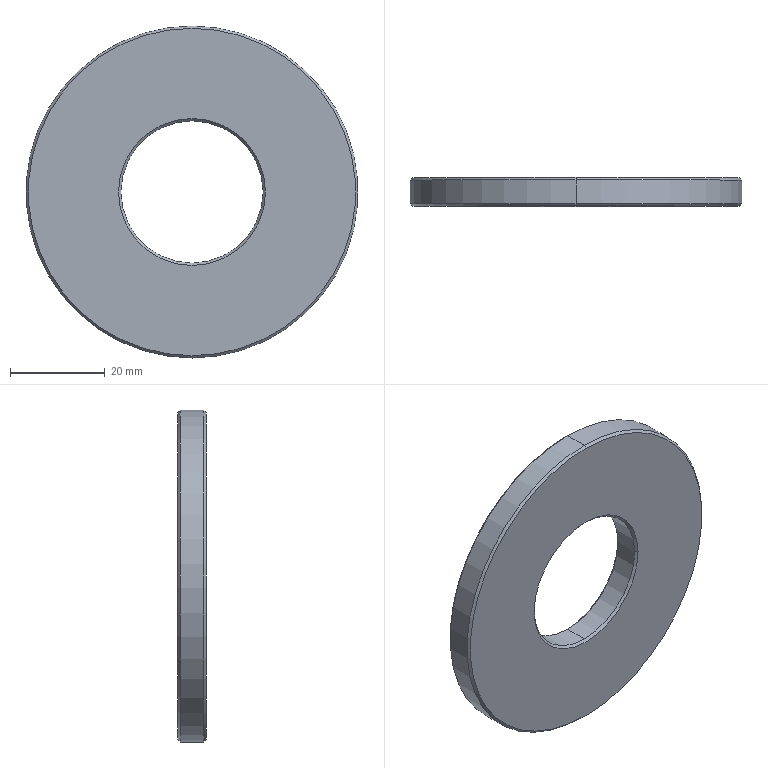Component | SolidWorks | YC1-250-04BalancerAssembly#16673-1_YC1-250-04-08Washer-1 | 1 solid | 14 faces | box 70 x 6 x 70 mm | volume 18771 mm3 | cone 8 | cylinder 4 | plane 2 | commonest cylinder face diameters 30 x2 70 x2 | material Plain Carbon Steel
STEP:
#1=COLOUR_RGB('',0.7922,0.8196,0.9333);
#2=FILL_AREA_STYLE_COLOUR('',#1);
#3=FILL_AREA_STYLE('',(#2));
#4=SURFACE_STYLE_FILL_AREA(#3);
#5=SURFACE_SIDE_STYLE('',(#4));
#6=SURFACE_STYLE_USAGE(.BOTH.,#5);
#7=PRESENTATION_STYLE_ASSIGNMENT((#6));
#8=CARTESIAN_POINT('',(-18.11,165.573,-0.5906));
#9=VERTEX_POINT('',#8);
#10=CARTESIAN_POINT('',(-18.11,165.573,0.5906));
#11=VERTEX_POINT('',#10);
#12=CARTESIAN_POINT('',(-18.11,165.573,-0.));
#13=DIRECTION('',(0.,1.,0.));
#14=DIRECTION('',(0.,0.,1.));
#15=AXIS2_PLACEMENT_3D('',#12,#13,#14);
#16=CIRCLE('',#15,0.5906);
#17=EDGE_CURVE('',#9,#11,#16,.T.);
#18=ORIENTED_EDGE('',*,*,#17,.F.);
#19=CARTESIAN_POINT('',(-18.11,165.592,-0.6102));
#20=VERTEX_POINT('',#19);
#21=CARTESIAN_POINT('',(-18.11,165.592,-0.6102));
#22=DIRECTION('',(0.,0.7071,-0.7071));
#23=VECTOR('',#22,39.37);
#24=LINE('',#21,#23);
#25=EDGE_CURVE('',#9,#20,#24,.T.);
#26=ORIENTED_EDGE('',*,*,#25,.T.);
#27=CARTESIAN_POINT('',(-18.11,165.592,0.6102));
#28=VERTEX_POINT('',#27);
#29=CARTESIAN_POINT('',(-18.11,165.592,-0.));
#30=DIRECTION('',(0.,-1.,0.));
#31=DIRECTION('',(0.,0.,1.));
#32=AXIS2_PLACEMENT_3D('',#29,#30,#31);
#33=CIRCLE('',#32,0.6102);
#34=EDGE_CURVE('',#28,#20,#33,.T.);
#35=ORIENTED_EDGE('',*,*,#34,.F.);
#36=CARTESIAN_POINT('',(-18.11,165.592,0.6102));
#37=DIRECTION('',(0.,0.7071,0.7071));
#38=VECTOR('',#37,39.37);
#39=LINE('',#36,#38);
#40=EDGE_CURVE('',#11,#28,#39,.T.);
#41=ORIENTED_EDGE('',*,*,#40,.F.);
#42=EDGE_LOOP('',(#18,#26,#35,#41));
#43=FACE_OUTER_BOUND('',#42,.T.);
#44=CARTESIAN_POINT('',(-18.11,165.592,-0.));
#45=DIRECTION('',(0.,1.,0.));
#46=DIRECTION('',(0.,0.,1.));
#47=AXIS2_PLACEMENT_3D('',#44,#45,#46);
#48=CONICAL_SURFACE('',#47,0.6102,0.7854);
#49=ADVANCED_FACE('',(#43),#48,.F.);
#50=CARTESIAN_POINT('',(-18.11,165.592,1.358));
#51=VERTEX_POINT('',#50);
#52=CARTESIAN_POINT('',(-18.11,165.592,-1.358));
#53=VERTEX_POINT('',#52);
#54=CARTESIAN_POINT('',(-18.11,165.592,-0.));
#55=DIRECTION('',(0.,1.,0.));
#56=DIRECTION('',(0.,0.,-1.));
#57=AXIS2_PLACEMENT_3D('',#54,#55,#56);
#58=CIRCLE('',#57,1.358);
#59=EDGE_CURVE('',#51,#53,#58,.T.);
#60=ORIENTED_EDGE('',*,*,#59,.F.);
#61=CARTESIAN_POINT('',(-18.11,165.573,1.378));
#62=VERTEX_POINT('',#61);
#63=CARTESIAN_POINT('',(-18.11,165.573,1.378));
#64=DIRECTION('',(0.,-0.7071,0.7071));
#65=VECTOR('',#64,39.37);
#66=LINE('',#63,#65);
#67=EDGE_CURVE('',#51,#62,#66,.T.);
#68=ORIENTED_EDGE('',*,*,#67,.T.);
#69=CARTESIAN_POINT('',(-18.11,165.573,-1.378));
#70=VERTEX_POINT('',#69);
#71=CARTESIAN_POINT('',(-18.11,165.573,-0.));
#72=DIRECTION('',(0.,1.,0.));
#73=DIRECTION('',(0.,0.,-1.));
#74=AXIS2_PLACEMENT_3D('',#71,#72,#73);
#75=CIRCLE('',#74,1.378);
#76=EDGE_CURVE('',#62,#70,#75,.T.);
#77=ORIENTED_EDGE('',*,*,#76,.T.);
#78=CARTESIAN_POINT('',(-18.11,165.573,-1.378));
#79=DIRECTION('',(0.,-0.7071,-0.7071));
#80=VECTOR('',#79,39.37);
#81=LINE('',#78,#80);
#82=EDGE_CURVE('',#53,#70,#81,.T.);
#83=ORIENTED_EDGE('',*,*,#82,.F.);
#84=EDGE_LOOP('',(#60,#68,#77,#83));
#85=FACE_OUTER_BOUND('',#84,.T.);
#86=CARTESIAN_POINT('',(-18.11,165.573,-0.));
#87=DIRECTION('',(0.,-1.,0.));
#88=DIRECTION('',(0.,0.,-1.));
#89=AXIS2_PLACEMENT_3D('',#86,#87,#88);
#90=CONICAL_SURFACE('',#89,1.378,0.7854);
#91=ADVANCED_FACE('',(#85),#90,.T.);
#92=ORIENTED_EDGE('',*,*,#17,.T.);
#93=CARTESIAN_POINT('',(-18.11,165.376,0.5906));
#94=VERTEX_POINT('',#93);
#95=CARTESIAN_POINT('',(-18.11,165.592,0.5906));
#96=DIRECTION('',(0.,-1.,0.));
#97=VECTOR('',#96,39.37);
#98=LINE('',#95,#97);
#99=EDGE_CURVE('',#11,#94,#98,.T.);
#100=ORIENTED_EDGE('',*,*,#99,.T.);
#101=CARTESIAN_POINT('',(-18.701,165.376,-0.));
#102=VERTEX_POINT('',#101);
#103=CARTESIAN_POINT('',(-18.11,165.376,-0.));
#104=DIRECTION('',(0.,1.,0.));
#105=DIRECTION('',(0.,0.,-1.));
#106=AXIS2_PLACEMENT_3D('',#103,#104,#105);
#107=CIRCLE('',#106,0.5906);
#108=EDGE_CURVE('',#102,#94,#107,.T.);
#109=ORIENTED_EDGE('',*,*,#108,.F.);
#110=CARTESIAN_POINT('',(-18.11,165.376,-0.5906));
#111=VERTEX_POINT('',#110);
#112=CARTESIAN_POINT('',(-18.11,165.376,-0.));
#113=DIRECTION('',(0.,1.,0.));
#114=DIRECTION('',(0.,0.,-1.));
#115=AXIS2_PLACEMENT_3D('',#112,#113,#114);
#116=CIRCLE('',#115,0.5906);
#117=EDGE_CURVE('',#111,#102,#116,.T.);
#118=ORIENTED_EDGE('',*,*,#117,.F.);
#119=CARTESIAN_POINT('',(-18.11,165.592,-0.5906));
#120=DIRECTION('',(0.,-1.,0.));
#121=VECTOR('',#120,39.37);
#122=LINE('',#119,#121);
#123=EDGE_CURVE('',#9,#111,#122,.T.);
#124=ORIENTED_EDGE('',*,*,#123,.F.);
#125=EDGE_LOOP('',(#92,#100,#109,#118,#124));
#126=FACE_OUTER_BOUND('',#125,.T.);
#127=CARTESIAN_POINT('',(-18.11,165.592,-0.));
#128=DIRECTION('',(0.,-1.,0.));
#129=DIRECTION('',(0.,0.,-1.));
#130=AXIS2_PLACEMENT_3D('',#127,#128,#129);
#131=CYLINDRICAL_SURFACE('',#130,0.5906);
#132=ADVANCED_FACE('',(#126),#131,.F.);
#133=ORIENTED_EDGE('',*,*,#76,.F.);
#134=CARTESIAN_POINT('',(-18.11,165.376,1.378));
#135=VERTEX_POINT('',#134);
#136=CARTESIAN_POINT('',(-18.11,165.592,1.378));
#137=DIRECTION('',(0.,-1.,0.));
#138=VECTOR('',#137,39.37);
#139=LINE('',#136,#138);
#140=EDGE_CURVE('',#62,#135,#139,.T.);
#141=ORIENTED_EDGE('',*,*,#140,.T.);
#142=CARTESIAN_POINT('',(-18.11,165.376,-1.378));
#143=VERTEX_POINT('',#142);
#144=CARTESIAN_POINT('',(-18.11,165.376,-0.));
#145=DIRECTION('',(0.,1.,0.));
#146=DIRECTION('',(0.,0.,-1.));
#147=AXIS2_PLACEMENT_3D('',#144,#145,#146);
#148=CIRCLE('',#147,1.378);
#149=EDGE_CURVE('',#135,#143,#148,.T.);
#150=ORIENTED_EDGE('',*,*,#149,.T.);
#151=CARTESIAN_POINT('',(-18.11,165.592,-1.378));
#152=DIRECTION('',(0.,-1.,0.));
#153=VECTOR('',#152,39.37);
#154=LINE('',#151,#153);
#155=EDGE_CURVE('',#70,#143,#154,.T.);
#156=ORIENTED_EDGE('',*,*,#155,.F.);
#157=EDGE_LOOP('',(#133,#141,#150,#156));
#158=FACE_OUTER_BOUND('',#157,.T.);
#159=CARTESIAN_POINT('',(-18.11,165.592,-0.));
#160=DIRECTION('',(0.,-1.,0.));
#161=DIRECTION('',(0.,0.,-1.));
#162=AXIS2_PLACEMENT_3D('',#159,#160,#161);
#163=CYLINDRICAL_SURFACE('',#162,1.378);
#164=ADVANCED_FACE('',(#158),#163,.T.);
#165=CARTESIAN_POINT('',(-17.52,165.376,-0.));
#166=VERTEX_POINT('',#165);
#167=CARTESIAN_POINT('',(-18.11,165.376,-0.));
#168=DIRECTION('',(0.,1.,0.));
#169=DIRECTION('',(0.,0.,-1.));
#170=AXIS2_PLACEMENT_3D('',#167,#168,#169);
#171=CIRCLE('',#170,0.5906);
#172=EDGE_CURVE('',#166,#111,#171,.T.);
#173=ORIENTED_EDGE('',*,*,#172,.T.);
#174=ORIENTED_EDGE('',*,*,#117,.T.);
#175=CARTESIAN_POINT('',(-18.72,165.356,-0.));
#176=VERTEX_POINT('',#175);
#177=CARTESIAN_POINT('',(-18.72,165.356,-0.));
#178=DIRECTION('',(-0.7071,-0.7071,0.));
#179=VECTOR('',#178,39.37);
#180=LINE('',#177,#179);
#181=EDGE_CURVE('',#102,#176,#180,.T.);
#182=ORIENTED_EDGE('',*,*,#181,.T.);
#183=CARTESIAN_POINT('',(-17.5,165.356,-0.));
#184=VERTEX_POINT('',#183);
#185=CARTESIAN_POINT('',(-18.11,165.356,-0.));
#186=DIRECTION('',(-0.,1.,0.));
#187=DIRECTION('',(1.,0.,0.));
#188=AXIS2_PLACEMENT_3D('',#185,#186,#187);
#189=CIRCLE('',#188,0.6102);
#190=EDGE_CURVE('',#184,#176,#189,.T.);
#191=ORIENTED_EDGE('',*,*,#190,.F.);
#192=CARTESIAN_POINT('',(-17.5,165.356,-0.));
#193=DIRECTION('',(0.7071,-0.7071,0.));
#194=VECTOR('',#193,39.37);
#195=LINE('',#192,#194);
#196=EDGE_CURVE('',#166,#184,#195,.T.);
#197=ORIENTED_EDGE('',*,*,#196,.F.);
#198=EDGE_LOOP('',(#173,#174,#182,#191,#197));
#199=FACE_OUTER_BOUND('',#198,.T.);
#200=CARTESIAN_POINT('',(-18.11,165.356,-0.));
#201=DIRECTION('',(0.,-1.,0.));
#202=DIRECTION('',(1.,0.,0.));
#203=AXIS2_PLACEMENT_3D('',#200,#201,#202);
#204=CONICAL_SURFACE('',#203,0.6102,0.7854);
#205=ADVANCED_FACE('',(#199),#204,.F.);
#206=CARTESIAN_POINT('',(-18.11,165.356,1.358));
#207=VERTEX_POINT('',#206);
#208=CARTESIAN_POINT('',(-18.11,165.356,-1.358));
#209=VERTEX_POINT('',#208);
#210=CARTESIAN_POINT('',(-18.11,165.356,-0.));
#211=DIRECTION('',(0.,1.,0.));
#212=DIRECTION('',(0.,0.,1.));
#213=AXIS2_PLACEMENT_3D('',#210,#211,#212);
#214=CIRCLE('',#213,1.358);
#215=EDGE_CURVE('',#207,#209,#214,.T.);
#216=ORIENTED_EDGE('',*,*,#215,.T.);
#217=CARTESIAN_POINT('',(-18.11,165.376,-1.378));
#218=DIRECTION('',(0.,0.7071,-0.7071));
#219=VECTOR('',#218,39.37);
#220=LINE('',#217,#219);
#221=EDGE_CURVE('',#209,#143,#220,.T.);
#222=ORIENTED_EDGE('',*,*,#221,.T.);
#223=ORIENTED_EDGE('',*,*,#149,.F.);
#224=CARTESIAN_POINT('',(-18.11,165.376,1.378));
#225=DIRECTION('',(0.,0.7071,0.7071));
#226=VECTOR('',#225,39.37);
#227=LINE('',#224,#226);
#228=EDGE_CURVE('',#207,#135,#227,.T.);
#229=ORIENTED_EDGE('',*,*,#228,.F.);
#230=EDGE_LOOP('',(#216,#222,#223,#229));
#231=FACE_OUTER_BOUND('',#230,.T.);
#232=CARTESIAN_POINT('',(-18.11,165.376,-0.));
#233=DIRECTION('',(0.,1.,0.));
#234=DIRECTION('',(0.,0.,1.));
#235=AXIS2_PLACEMENT_3D('',#232,#233,#234);
#236=CONICAL_SURFACE('',#235,1.378,0.7854);
#237=ADVANCED_FACE('',(#231),#236,.T.);
#238=ORIENTED_EDGE('',*,*,#34,.T.);
#239=CARTESIAN_POINT('',(-18.11,165.592,-0.));
#240=DIRECTION('',(0.,-1.,0.));
#241=DIRECTION('',(0.,0.,1.));
#242=AXIS2_PLACEMENT_3D('',#239,#240,#241);
#243=CIRCLE('',#242,0.6102);
#244=EDGE_CURVE('',#20,#28,#243,.T.);
#245=ORIENTED_EDGE('',*,*,#244,.T.);
#246=EDGE_LOOP('',(#238,#245));
#247=FACE_BOUND('',#246,.T.);
#248=CARTESIAN_POINT('',(-18.11,165.592,-0.));
#249=DIRECTION('',(0.,1.,0.));
#250=DIRECTION('',(0.,0.,-1.));
#251=AXIS2_PLACEMENT_3D('',#248,#249,#250);
#252=CIRCLE('',#251,1.358);
#253=EDGE_CURVE('',#53,#51,#252,.T.);
#254=ORIENTED_EDGE('',*,*,#253,.T.);
#255=ORIENTED_EDGE('',*,*,#59,.T.);
#256=EDGE_LOOP('',(#254,#255));
#257=FACE_OUTER_BOUND('',#256,.T.);
#258=CARTESIAN_POINT('',(-18.11,165.592,-0.));
#259=DIRECTION('',(0.,1.,0.));
#260=DIRECTION('',(0.,0.,1.));
#261=AXIS2_PLACEMENT_3D('',#258,#259,#260);
#262=PLANE('',#261);
#263=ADVANCED_FACE('',(#247,#257),#262,.T.);
#264=ORIENTED_EDGE('',*,*,#25,.F.);
#265=CARTESIAN_POINT('',(-18.11,165.573,-0.));
#266=DIRECTION('',(0.,1.,0.));
#267=DIRECTION('',(0.,0.,1.));
#268=AXIS2_PLACEMENT_3D('',#265,#266,#267);
#269=CIRCLE('',#268,0.5906);
#270=EDGE_CURVE('',#11,#9,#269,.T.);
#271=ORIENTED_EDGE('',*,*,#270,.F.);
#272=ORIENTED_EDGE('',*,*,#40,.T.);
#273=ORIENTED_EDGE('',*,*,#244,.F.);
#274=EDGE_LOOP('',(#264,#271,#272,#273));
#275=FACE_OUTER_BOUND('',#274,.T.);
#276=CARTESIAN_POINT('',(-18.11,165.592,-0.));
#277=DIRECTION('',(0.,1.,0.));
#278=DIRECTION('',(0.,0.,1.));
#279=AXIS2_PLACEMENT_3D('',#276,#277,#278);
#280=CONICAL_SURFACE('',#279,0.6102,0.7854);
#281=ADVANCED_FACE('',(#275),#280,.F.);
#282=ORIENTED_EDGE('',*,*,#67,.F.);
#283=ORIENTED_EDGE('',*,*,#253,.F.);
#284=ORIENTED_EDGE('',*,*,#82,.T.);
#285=CARTESIAN_POINT('',(-18.11,165.573,-0.));
#286=DIRECTION('',(0.,1.,0.));
#287=DIRECTION('',(0.,0.,-1.));
#288=AXIS2_PLACEMENT_3D('',#285,#286,#287);
#289=CIRCLE('',#288,1.378);
#290=EDGE_CURVE('',#70,#62,#289,.T.);
#291=ORIENTED_EDGE('',*,*,#290,.T.);
#292=EDGE_LOOP('',(#282,#283,#284,#291));
#293=FACE_OUTER_BOUND('',#292,.T.);
#294=CARTESIAN_POINT('',(-18.11,165.573,-0.));
#295=DIRECTION('',(0.,-1.,0.));
#296=DIRECTION('',(0.,0.,-1.));
#297=AXIS2_PLACEMENT_3D('',#294,#295,#296);
#298=CONICAL_SURFACE('',#297,1.378,0.7854);
#299=ADVANCED_FACE('',(#293),#298,.T.);
#300=ORIENTED_EDGE('',*,*,#99,.F.);
#301=ORIENTED_EDGE('',*,*,#270,.T.);
#302=ORIENTED_EDGE('',*,*,#123,.T.);
#303=ORIENTED_EDGE('',*,*,#172,.F.);
#304=CARTESIAN_POINT('',(-18.11,165.376,-0.));
#305=DIRECTION('',(0.,1.,0.));
#306=DIRECTION('',(0.,0.,-1.));
#307=AXIS2_PLACEMENT_3D('',#304,#305,#306);
#308=CIRCLE('',#307,0.5906);
#309=EDGE_CURVE('',#94,#166,#308,.T.);
#310=ORIENTED_EDGE('',*,*,#309,.F.);
#311=EDGE_LOOP('',(#300,#301,#302,#303,#310));
#312=FACE_OUTER_BOUND('',#311,.T.);
#313=CARTESIAN_POINT('',(-18.11,165.592,-0.));
#314=DIRECTION('',(0.,-1.,0.));
#315=DIRECTION('',(0.,0.,-1.));
#316=AXIS2_PLACEMENT_3D('',#313,#314,#315);
#317=CYLINDRICAL_SURFACE('',#316,0.5906);
#318=ADVANCED_FACE('',(#312),#317,.F.);
#319=ORIENTED_EDGE('',*,*,#140,.F.);
#320=ORIENTED_EDGE('',*,*,#290,.F.);
#321=ORIENTED_EDGE('',*,*,#155,.T.);
#322=CARTESIAN_POINT('',(-18.11,165.376,-0.));
#323=DIRECTION('',(0.,1.,0.));
#324=DIRECTION('',(0.,0.,-1.));
#325=AXIS2_PLACEMENT_3D('',#322,#323,#324);
#326=CIRCLE('',#325,1.378);
#327=EDGE_CURVE('',#143,#135,#326,.T.);
#328=ORIENTED_EDGE('',*,*,#327,.T.);
#329=EDGE_LOOP('',(#319,#320,#321,#328));
#330=FACE_OUTER_BOUND('',#329,.T.);
#331=CARTESIAN_POINT('',(-18.11,165.592,-0.));
#332=DIRECTION('',(0.,-1.,0.));
#333=DIRECTION('',(0.,0.,-1.));
#334=AXIS2_PLACEMENT_3D('',#331,#332,#333);
#335=CYLINDRICAL_SURFACE('',#334,1.378);
#336=ADVANCED_FACE('',(#330),#335,.T.);
#337=ORIENTED_EDGE('',*,*,#181,.F.);
#338=ORIENTED_EDGE('',*,*,#108,.T.);
#339=ORIENTED_EDGE('',*,*,#309,.T.);
#340=ORIENTED_EDGE('',*,*,#196,.T.);
#341=CARTESIAN_POINT('',(-18.11,165.356,-0.));
#342=DIRECTION('',(-0.,1.,0.));
#343=DIRECTION('',(1.,0.,0.));
#344=AXIS2_PLACEMENT_3D('',#341,#342,#343);
#345=CIRCLE('',#344,0.6102);
#346=EDGE_CURVE('',#176,#184,#345,.T.);
#347=ORIENTED_EDGE('',*,*,#346,.F.);
#348=EDGE_LOOP('',(#337,#338,#339,#340,#347));
#349=FACE_OUTER_BOUND('',#348,.T.);
#350=CARTESIAN_POINT('',(-18.11,165.356,-0.));
#351=DIRECTION('',(0.,-1.,0.));
#352=DIRECTION('',(1.,0.,0.));
#353=AXIS2_PLACEMENT_3D('',#350,#351,#352);
#354=CONICAL_SURFACE('',#353,0.6102,0.7854);
#355=ADVANCED_FACE('',(#349),#354,.F.);
#356=ORIENTED_EDGE('',*,*,#221,.F.);
#357=CARTESIAN_POINT('',(-18.11,165.356,-0.));
#358=DIRECTION('',(0.,1.,0.));
#359=DIRECTION('',(0.,0.,1.));
#360=AXIS2_PLACEMENT_3D('',#357,#358,#359);
#361=CIRCLE('',#360,1.358);
#362=EDGE_CURVE('',#209,#207,#361,.T.);
#363=ORIENTED_EDGE('',*,*,#362,.T.);
#364=ORIENTED_EDGE('',*,*,#228,.T.);
#365=ORIENTED_EDGE('',*,*,#327,.F.);
#366=EDGE_LOOP('',(#356,#363,#364,#365));
#367=FACE_OUTER_BOUND('',#366,.T.);
#368=CARTESIAN_POINT('',(-18.11,165.376,-0.));
#369=DIRECTION('',(0.,1.,0.));
#370=DIRECTION('',(0.,0.,1.));
#371=AXIS2_PLACEMENT_3D('',#368,#369,#370);
#372=CONICAL_SURFACE('',#371,1.378,0.7854);
#373=ADVANCED_FACE('',(#367),#372,.T.);
#374=ORIENTED_EDGE('',*,*,#190,.T.);
#375=ORIENTED_EDGE('',*,*,#346,.T.);
#376=EDGE_LOOP('',(#374,#375));
#377=FACE_BOUND('',#376,.T.);
#378=ORIENTED_EDGE('',*,*,#215,.F.);
#379=ORIENTED_EDGE('',*,*,#362,.F.);
#380=EDGE_LOOP('',(#378,#379));
#381=FACE_OUTER_BOUND('',#380,.T.);
#382=CARTESIAN_POINT('',(-18.11,165.356,-0.));
#383=DIRECTION('',(0.,1.,0.));
#384=DIRECTION('',(0.,0.,1.));
#385=AXIS2_PLACEMENT_3D('',#382,#383,#384);
#386=PLANE('',#385);
#387=ADVANCED_FACE('',(#377,#381),#386,.F.);
#388=CLOSED_SHELL('',(#49,#91,#132,#164,#205,#237,#263,#281,#299,#318,#336,#355,#373,#387));
#389=MANIFOLD_SOLID_BREP('',#388);
#390=STYLED_ITEM('',(#7),#389);
#391=(LENGTH_UNIT()NAMED_UNIT(*)SI_UNIT($,.METRE.));
#392=LENGTH_MEASURE_WITH_UNIT(LENGTH_MEASURE(0.0254),#391);
#393=DIMENSIONAL_EXPONENTS(1.,0.,0.,0.,0.,0.,0.);
#394=(CONVERSION_BASED_UNIT('',#392)LENGTH_UNIT()NAMED_UNIT(#393));
#395=UNCERTAINTY_MEASURE_WITH_UNIT(LENGTH_MEASURE(0.00001),#394,'','');
#396=(NAMED_UNIT(*)PLANE_ANGLE_UNIT()SI_UNIT($,.RADIAN.));
#397=(NAMED_UNIT(*)SI_UNIT($,.STERADIAN.)SOLID_ANGLE_UNIT());
#398=(GEOMETRIC_REPRESENTATION_CONTEXT(3)GLOBAL_UNCERTAINTY_ASSIGNED_CONTEXT((#395))GLOBAL_UNIT_ASSIGNED_CONTEXT((#394,#396,#397))REPRESENTATION_CONTEXT('',''));
#399=MECHANICAL_DESIGN_GEOMETRIC_PRESENTATION_REPRESENTATION('',(#390),#398);
#400=CARTESIAN_POINT('',(0.,0.,0.));
#401=DIRECTION('',(0.,0.,1.));
#402=DIRECTION('',(1.,0.,0.));
#403=AXIS2_PLACEMENT_3D('',#400,#401,#402);
#404=(LENGTH_UNIT()NAMED_UNIT(*)SI_UNIT($,.METRE.));
#405=LENGTH_MEASURE_WITH_UNIT(LENGTH_MEASURE(0.0254),#404);
#406=DIMENSIONAL_EXPONENTS(1.,0.,0.,0.,0.,0.,0.);
#407=(CONVERSION_BASED_UNIT('',#405)LENGTH_UNIT()NAMED_UNIT(#406));
#408=UNCERTAINTY_MEASURE_WITH_UNIT(LENGTH_MEASURE(0.00001),#407,'','');
#409=(NAMED_UNIT(*)PLANE_ANGLE_UNIT()SI_UNIT($,.RADIAN.));
#410=(NAMED_UNIT(*)SI_UNIT($,.STERADIAN.)SOLID_ANGLE_UNIT());
#411=(GEOMETRIC_REPRESENTATION_CONTEXT(3)GLOBAL_UNCERTAINTY_ASSIGNED_CONTEXT((#408))GLOBAL_UNIT_ASSIGNED_CONTEXT((#407,#409,#410))REPRESENTATION_CONTEXT('',''));
#412=ADVANCED_BREP_SHAPE_REPRESENTATION('',(#389,#403),#411);
#413=PRESENTATION_LAYER_ASSIGNMENT('','',(#390));